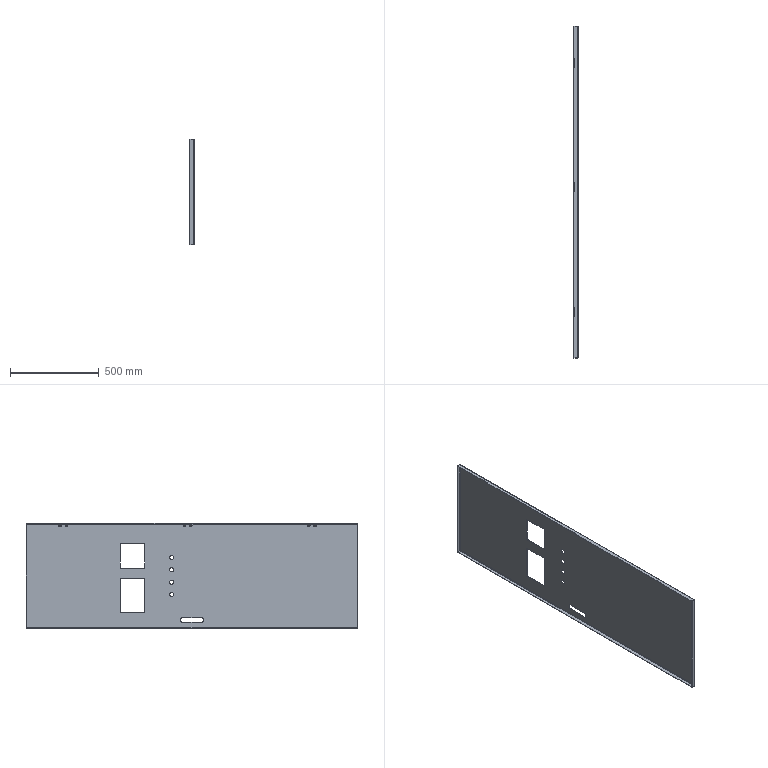Component | SolidWorks | LeftFrontDoorAssembly-1_LeftFrontDoorPanel07-01-1 | 1 solid | 98 faces | volume 2314942 mm3 | plane 46 | cylinder 44 | spline 8 | commonest cylinder face diameters 6 x28 23 x8 5 x4 9 x4